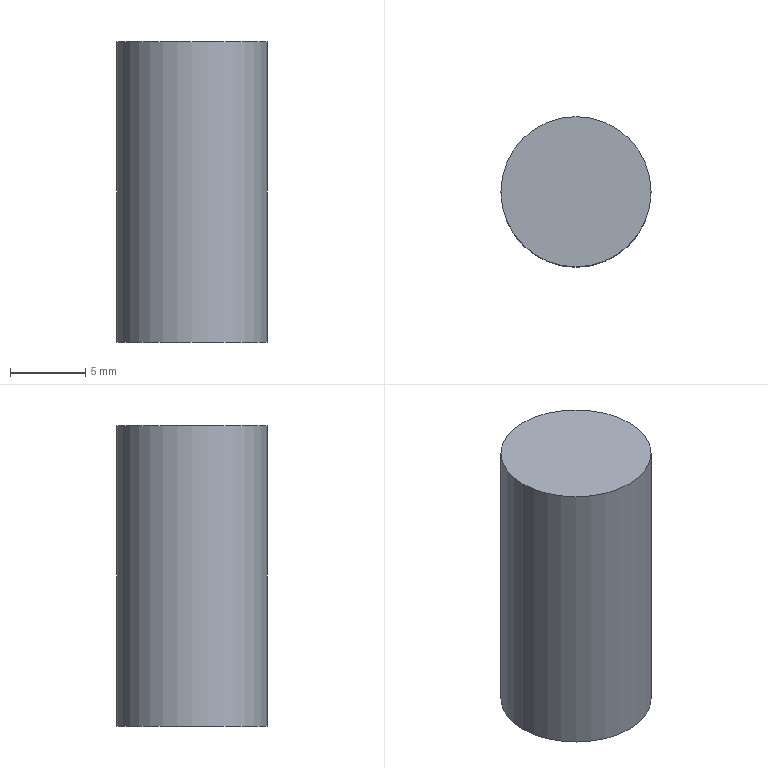Component | NX | PINO_BASE4FURO_2 | 1 solid | 3 faces | box 10 x 10 x 20 mm | volume 1571 mm3 | plane 2 | cylinder 1 | commonest cylinder face diameters 10 x1
STEP:
#1=CARTESIAN_POINT('',(0.,0.,0.));
#2=DIRECTION('',(0.,0.,1.));
#3=DIRECTION('',(1.,0.,0.));
#4=AXIS2_PLACEMENT_3D('',#1,#2,#3);
#5=CARTESIAN_POINT('',(-53.,30.,40.));
#6=VERTEX_POINT('',#5);
#7=CARTESIAN_POINT('',(-58.,30.,40.));
#8=DIRECTION('',(0.,0.,-1.));
#9=DIRECTION('',(1.,0.,0.));
#10=AXIS2_PLACEMENT_3D('',#7,#8,#9);
#11=CIRCLE('',#10,5.);
#12=CARTESIAN_POINT('',(-58.,30.,40.));
#13=DIRECTION('',(0.,0.,1.));
#14=DIRECTION('',(-1.,0.,0.));
#15=AXIS2_PLACEMENT_3D('',#12,#13,#14);
#16=CYLINDRICAL_SURFACE('',#15,5.);
#17=CARTESIAN_POINT('',(9.425,0.));
#18=DIRECTION('',(-1.,0.));
#19=VECTOR('',#18,1.);
#20=LINE('',#17,#19);
#21=(GEOMETRIC_REPRESENTATION_CONTEXT(2)PARAMETRIC_REPRESENTATION_CONTEXT()REPRESENTATION_CONTEXT('',''));
#22=DEFINITIONAL_REPRESENTATION('',(#20),#21);
#23=PCURVE('',#16,#22);
#24=CARTESIAN_POINT('',(-58.,30.,40.));
#25=DIRECTION('',(0.,0.,-1.));
#26=DIRECTION('',(1.,0.,0.));
#27=AXIS2_PLACEMENT_3D('',#24,#25,#26);
#28=PLANE('',#27);
#29=CARTESIAN_POINT('',(0.,0.));
#30=DIRECTION('',(1.,0.));
#31=AXIS2_PLACEMENT_2D('',#29,#30);
#32=CIRCLE('',#31,5.);
#33=(GEOMETRIC_REPRESENTATION_CONTEXT(2)PARAMETRIC_REPRESENTATION_CONTEXT()REPRESENTATION_CONTEXT('',''));
#34=DEFINITIONAL_REPRESENTATION('',(#32),#33);
#35=PCURVE('',#28,#34);
#36=SURFACE_CURVE('',#11,(#23,#35),.PCURVE_S1.);
#37=EDGE_CURVE('',#6,#6,#36,.T.);
#38=ORIENTED_EDGE('',*,*,#37,.F.);
#39=CARTESIAN_POINT('',(-53.,30.,60.));
#40=VERTEX_POINT('',#39);
#41=CARTESIAN_POINT('',(-53.,30.,40.));
#42=CARTESIAN_POINT('',(-53.,30.,60.));
#43=B_SPLINE_CURVE_WITH_KNOTS('',1,(#41,#42),.UNSPECIFIED.,.F.,.F.,(2,2),(0.,20.),.PIECEWISE_BEZIER_KNOTS.);
#44=CARTESIAN_POINT('',(9.425,0.));
#45=DIRECTION('',(0.,1.));
#46=VECTOR('',#45,1.);
#47=LINE('',#44,#46);
#48=(GEOMETRIC_REPRESENTATION_CONTEXT(2)PARAMETRIC_REPRESENTATION_CONTEXT()REPRESENTATION_CONTEXT('',''));
#49=DEFINITIONAL_REPRESENTATION('',(#47),#48);
#50=PCURVE('',#16,#49);
#51=CARTESIAN_POINT('',(3.142,0.));
#52=DIRECTION('',(0.,1.));
#53=VECTOR('',#52,1.);
#54=LINE('',#51,#53);
#55=(GEOMETRIC_REPRESENTATION_CONTEXT(2)PARAMETRIC_REPRESENTATION_CONTEXT()REPRESENTATION_CONTEXT('',''));
#56=DEFINITIONAL_REPRESENTATION('',(#54),#55);
#57=PCURVE('',#16,#56);
#58=SEAM_CURVE('',#43,(#50,#57),.PCURVE_S1.);
#59=EDGE_CURVE('',#6,#40,#58,.T.);
#60=ORIENTED_EDGE('',*,*,#59,.T.);
#61=CARTESIAN_POINT('',(-58.,30.,60.));
#62=DIRECTION('',(0.,0.,-1.));
#63=DIRECTION('',(1.,0.,0.));
#64=AXIS2_PLACEMENT_3D('',#61,#62,#63);
#65=CIRCLE('',#64,5.);
#66=CARTESIAN_POINT('',(9.425,20.));
#67=DIRECTION('',(-1.,0.));
#68=VECTOR('',#67,1.);
#69=LINE('',#66,#68);
#70=(GEOMETRIC_REPRESENTATION_CONTEXT(2)PARAMETRIC_REPRESENTATION_CONTEXT()REPRESENTATION_CONTEXT('',''));
#71=DEFINITIONAL_REPRESENTATION('',(#69),#70);
#72=PCURVE('',#16,#71);
#73=CARTESIAN_POINT('',(-58.,30.,60.));
#74=DIRECTION('',(0.,0.,-1.));
#75=DIRECTION('',(1.,0.,0.));
#76=AXIS2_PLACEMENT_3D('',#73,#74,#75);
#77=PLANE('',#76);
#78=CARTESIAN_POINT('',(0.,0.));
#79=DIRECTION('',(1.,0.));
#80=AXIS2_PLACEMENT_2D('',#78,#79);
#81=CIRCLE('',#80,5.);
#82=(GEOMETRIC_REPRESENTATION_CONTEXT(2)PARAMETRIC_REPRESENTATION_CONTEXT()REPRESENTATION_CONTEXT('',''));
#83=DEFINITIONAL_REPRESENTATION('',(#81),#82);
#84=PCURVE('',#77,#83);
#85=SURFACE_CURVE('',#65,(#72,#84),.PCURVE_S1.);
#86=EDGE_CURVE('',#40,#40,#85,.T.);
#87=ORIENTED_EDGE('',*,*,#86,.T.);
#88=ORIENTED_EDGE('',*,*,#59,.F.);
#89=EDGE_LOOP('',(#38,#60,#87,#88));
#90=FACE_BOUND('',#89,.T.);
#91=ADVANCED_FACE('',(#90),#16,.T.);
#92=ORIENTED_EDGE('',*,*,#37,.T.);
#93=EDGE_LOOP('',(#92));
#94=FACE_BOUND('',#93,.T.);
#95=ADVANCED_FACE('',(#94),#28,.T.);
#96=ORIENTED_EDGE('',*,*,#86,.F.);
#97=EDGE_LOOP('',(#96));
#98=FACE_BOUND('',#97,.T.);
#99=ADVANCED_FACE('',(#98),#77,.F.);
#100=CLOSED_SHELL('',(#91,#95,#99));
#101=MANIFOLD_SOLID_BREP('',#100);
#102=(LENGTH_UNIT()NAMED_UNIT(*)SI_UNIT(.MILLI.,.METRE.));
#103=UNCERTAINTY_MEASURE_WITH_UNIT(LENGTH_MEASURE(0.00001),#102,'','');
#104=(NAMED_UNIT(*)PLANE_ANGLE_UNIT()SI_UNIT($,.RADIAN.));
#105=(NAMED_UNIT(*)SI_UNIT($,.STERADIAN.)SOLID_ANGLE_UNIT());
#106=(GEOMETRIC_REPRESENTATION_CONTEXT(3)GLOBAL_UNCERTAINTY_ASSIGNED_CONTEXT((#103))GLOBAL_UNIT_ASSIGNED_CONTEXT((#102,#104,#105))REPRESENTATION_CONTEXT('',''));
#107=ADVANCED_BREP_SHAPE_REPRESENTATION('',(#4,#101),#106);